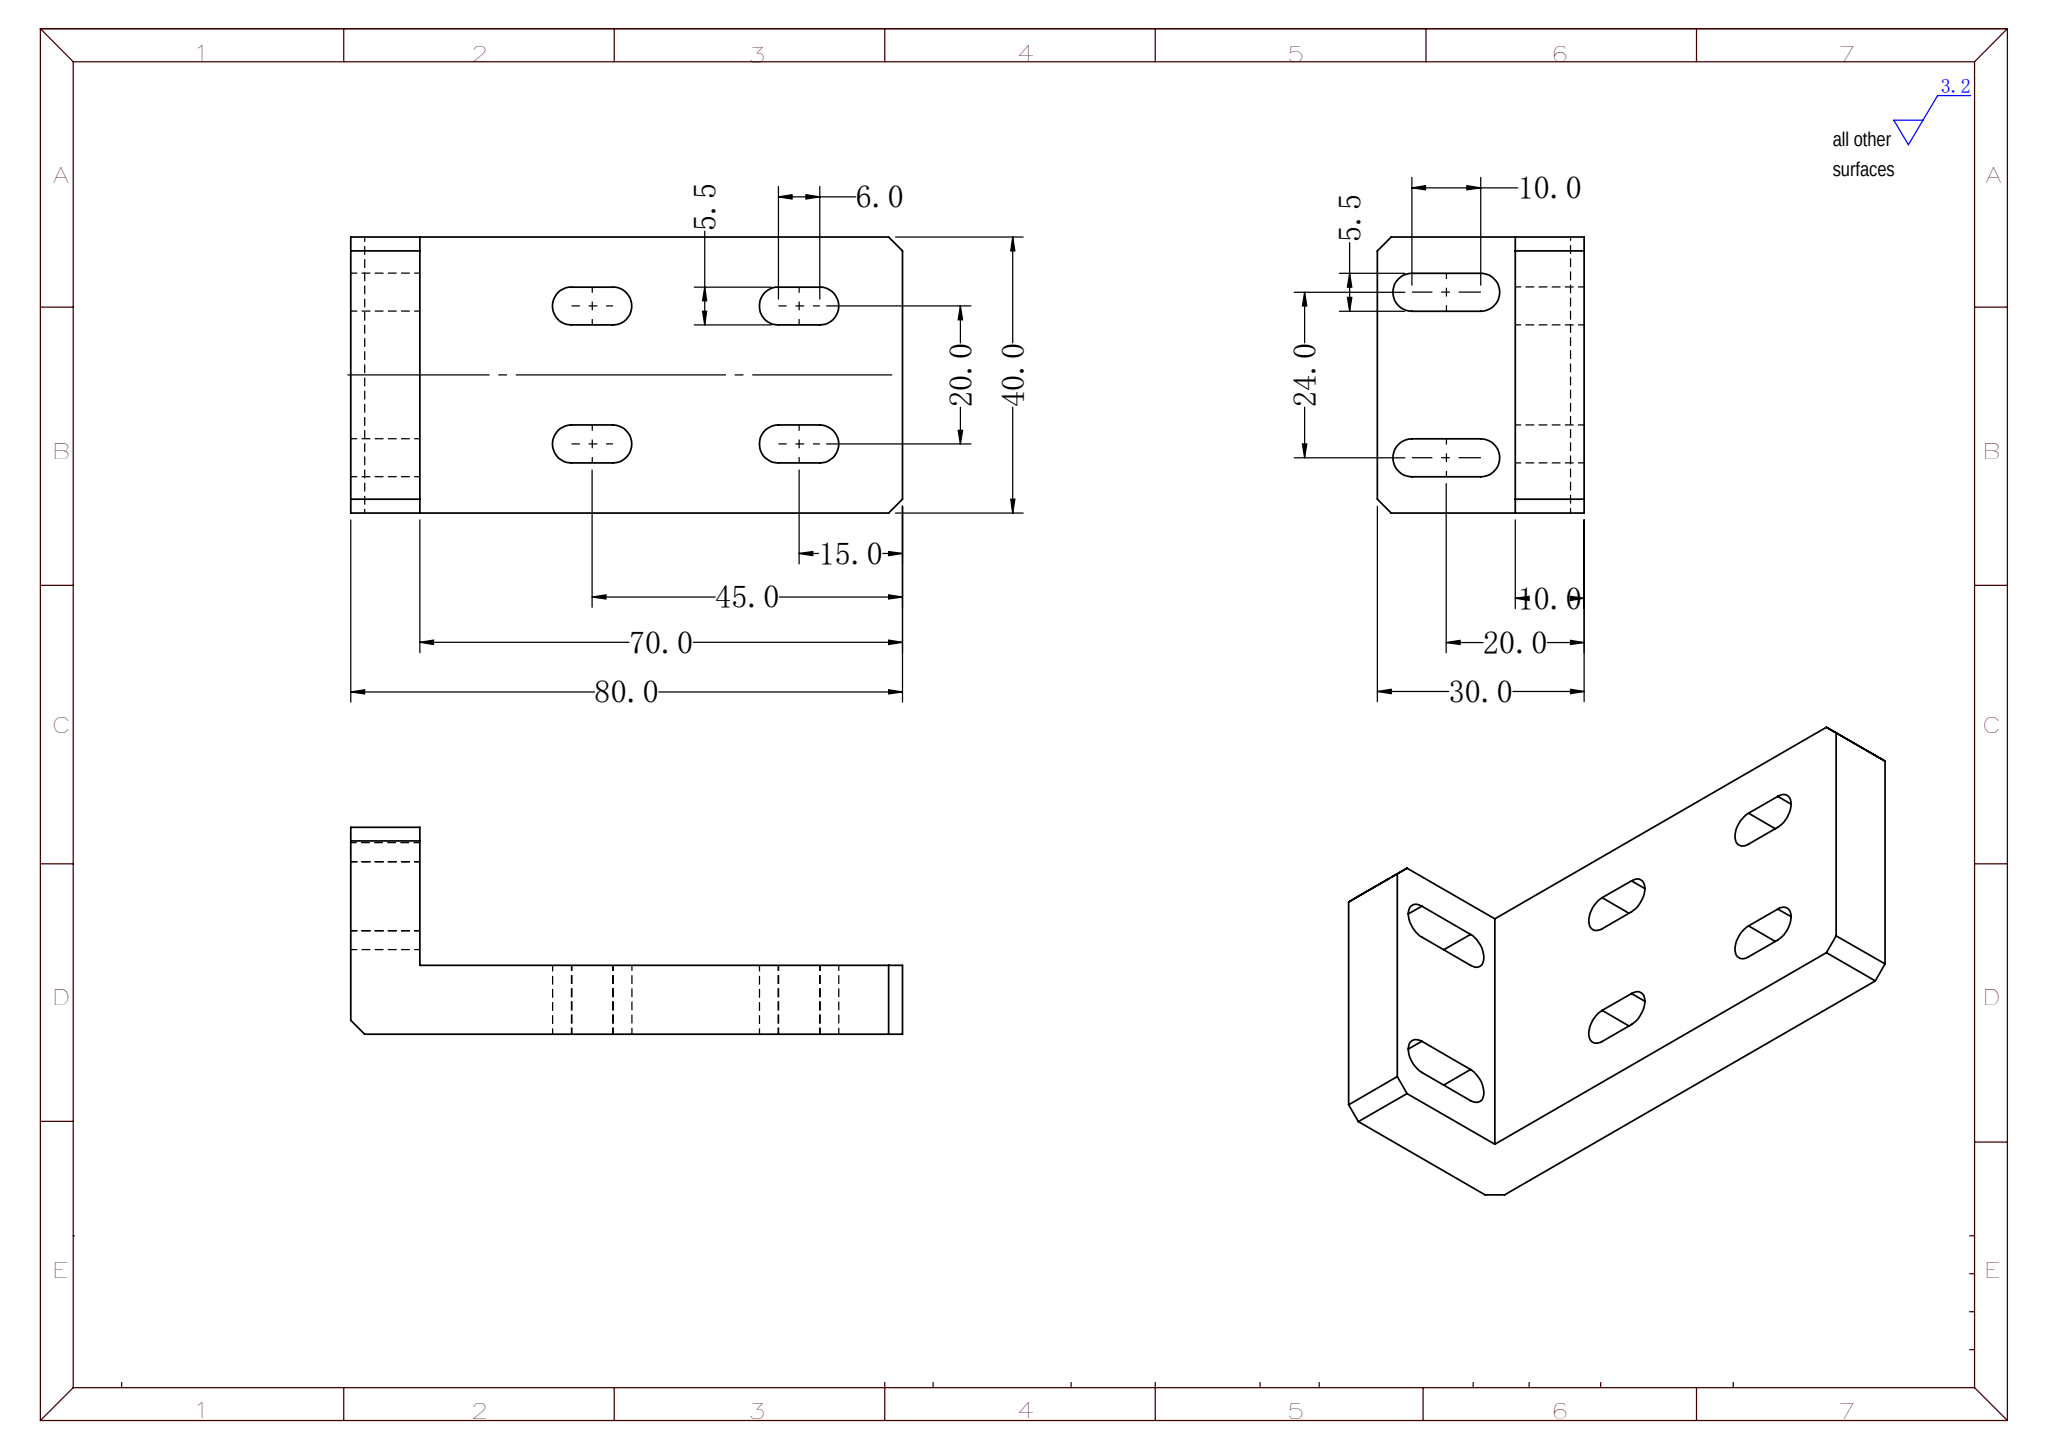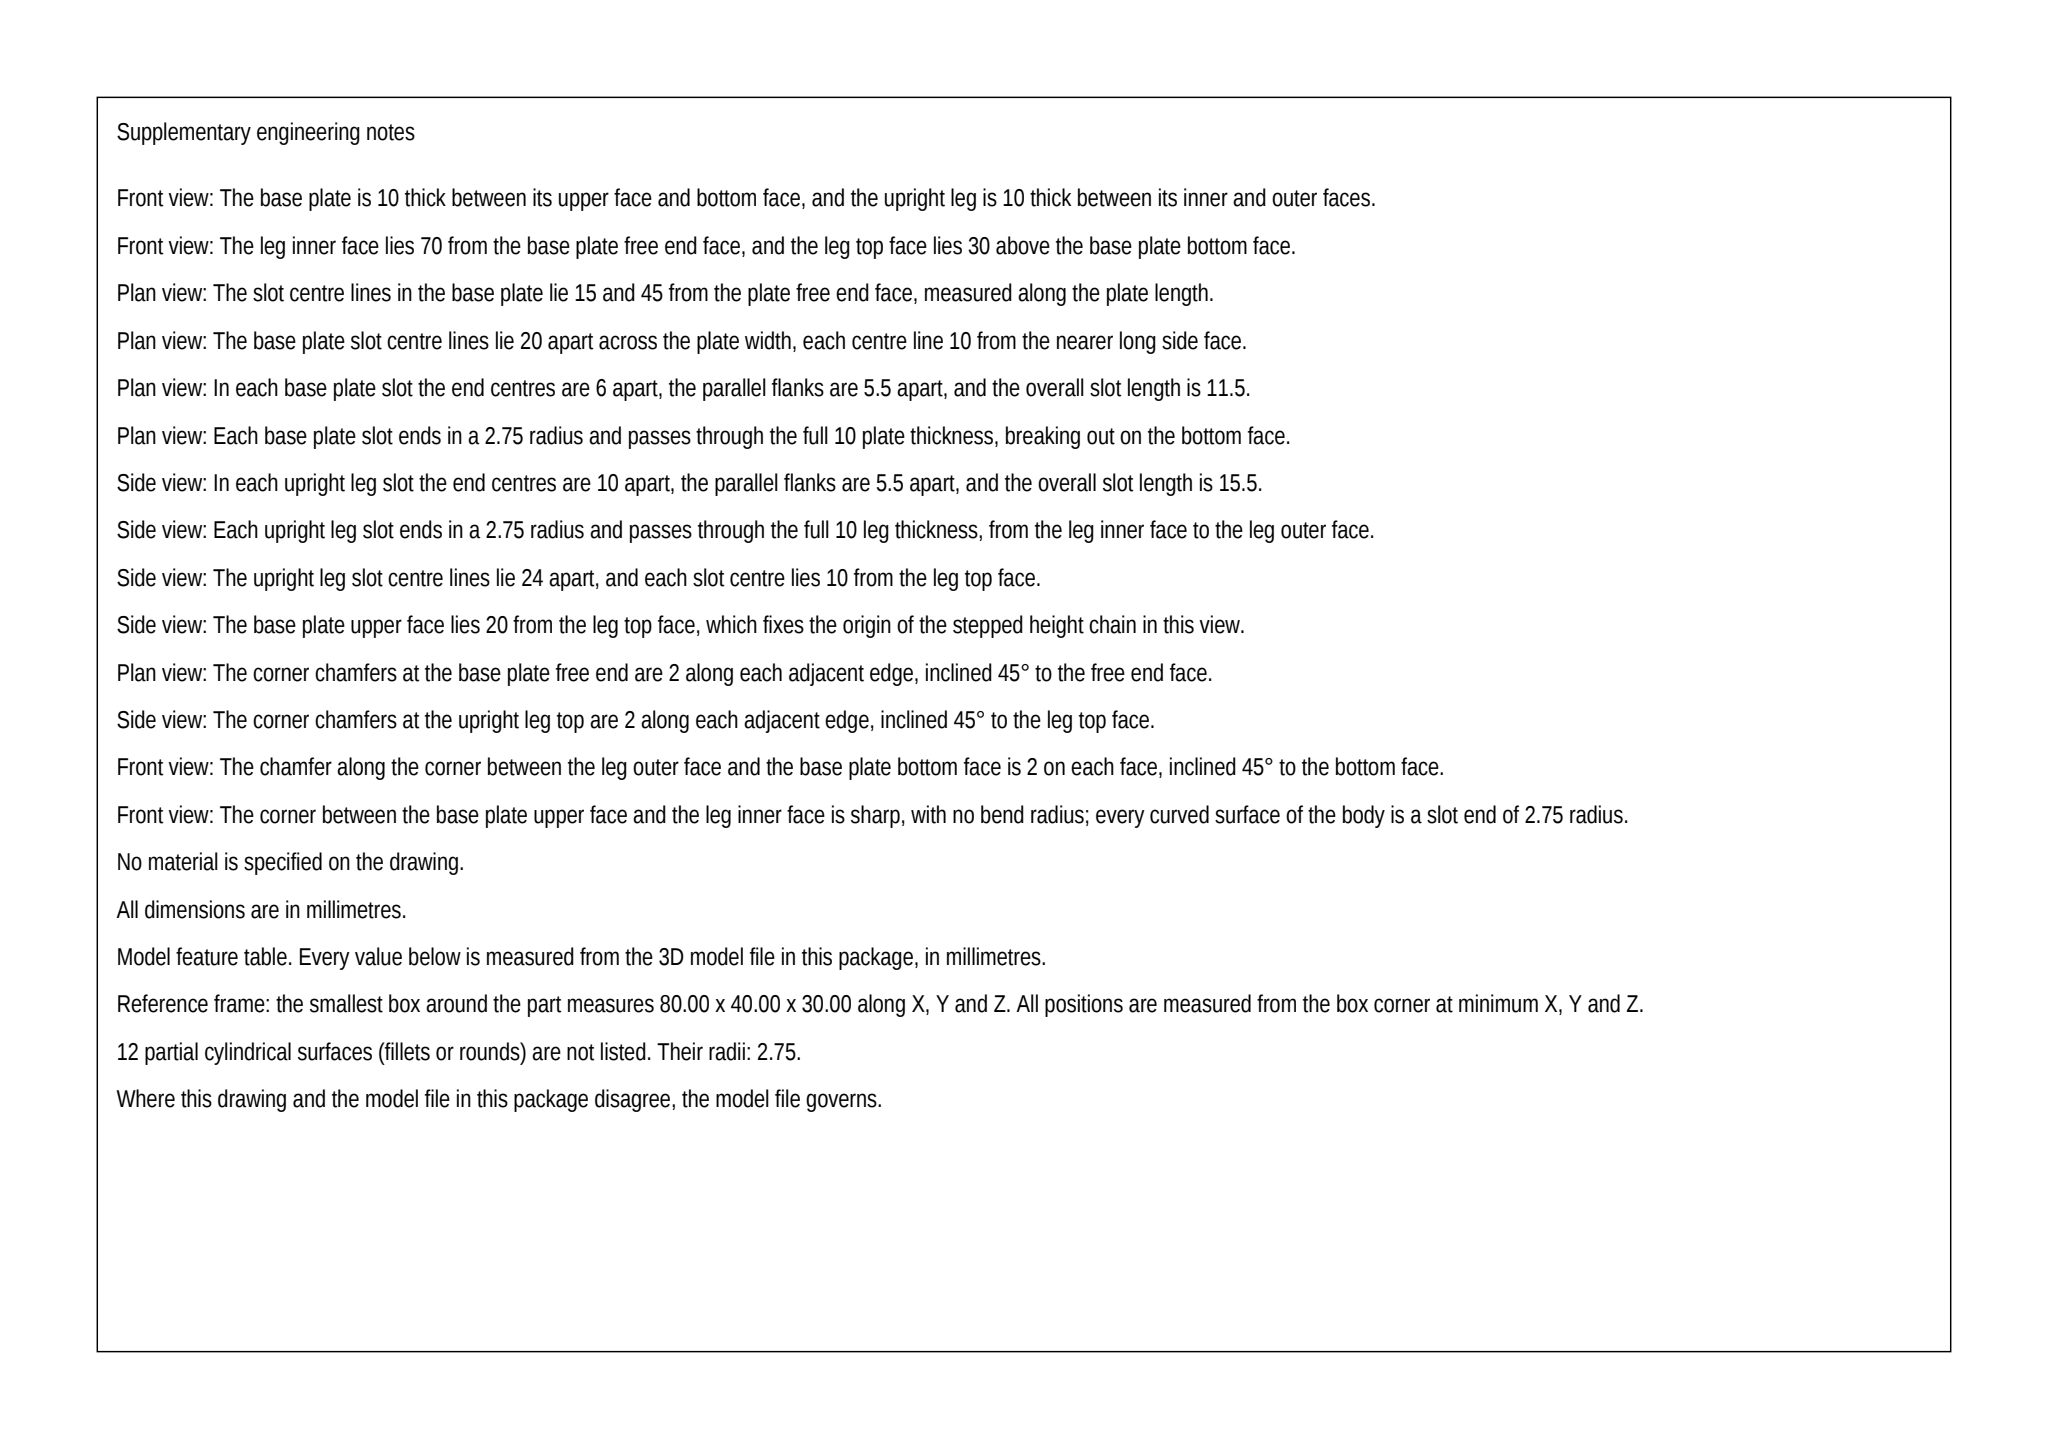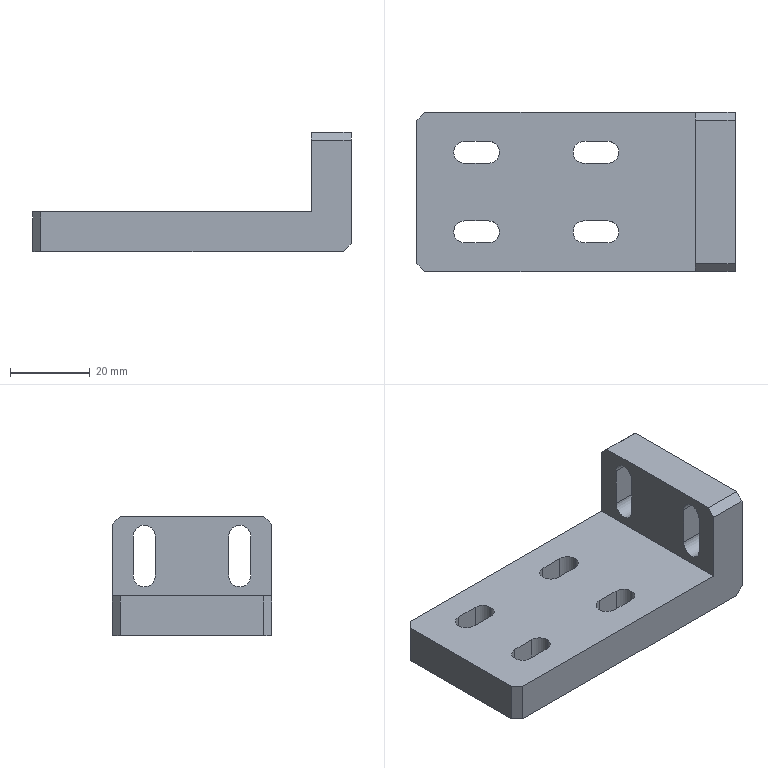Part | SolidWorks | mm | 1 solid | 43 faces | box 80 x 40 x 30 mm | volume 35995 mm3 | plane 25 | cylinder 18 | commonest cylinder face diameters 5.5 x18
Drawing notes:
ALL CORNERS C5 (5 x 45°) - PLATE END & UPRIGHT LEG | from the solid: BBox 80x40x30; corner cuts at x=0 plate end and leg top (z=30) are 45° planes, not in axis_planes list; measured leg 5 mm each side in TOP & SIDE views
build123d program:
from build123d import *

# Parameters (mm, degrees)
SKETCH1_W           = 80
SKETCH1_H           = 40
BOSS_EXTRUDE1_DEPTH = 15
SKETCH2_W           = 70
SKETCH2_H           = 20
CUT_EXTRUDE1_DEPTH  = 59.523
CUT_EXTRUDE2_DEPTH  = 75.33
CUT_EXTRUDE3_DEPTH  = 49.99
CHAMFER1_SIZE       = 2


with BuildPart() as part:
    # Sketch1 → Boss-Extrude1 (new, symmetric)
    with BuildSketch(Plane.XY):
        Rectangle(SKETCH1_W, SKETCH1_H)
    extrude(amount=BOSS_EXTRUDE1_DEPTH, both=True)

    # Sketch2 → Cut-Extrude1 (cut, through all)
    with BuildSketch(Plane(origin=(0, 20, 0), x_dir=(1, 0, 0), z_dir=(0, 1, 0))):
        with Locations((-5, -5)):
            Rectangle(SKETCH2_W, SKETCH2_H)
    extrude(amount=-CUT_EXTRUDE1_DEPTH, mode=Mode.SUBTRACT)

    # Sketch3 → Cut-Extrude2 (cut, through all)
    with BuildSketch(Plane.ZY.offset(-30)):
        with BuildLine():
            Line((0, 14.75), (10, 14.75))
            ThreePointArc((10, 14.75), (12.75, 12), (10, 9.25))
            Line((10, 9.25), (0, 9.25))
            ThreePointArc((0, 9.25), (-2.75, 12), (0, 14.75))
        make_face()
        with BuildLine():
            Line((0, -14.75), (10, -14.75))
            ThreePointArc((10, -14.75), (12.75, -12), (10, -9.25))
            Line((10, -9.25), (0, -9.25))
            ThreePointArc((0, -9.25), (-2.75, -12), (0, -14.75))
        make_face()
    extrude(amount=-CUT_EXTRUDE2_DEPTH, mode=Mode.SUBTRACT)

    # Sketch4 → Cut-Extrude3 (cut, through all)
    with BuildSketch(Plane.XY.offset(-5)):
        with BuildLine():
            Line((-28, 12.75), (-22, 12.75))
            ThreePointArc((-22, 12.75), (-19.25, 10), (-22, 7.25))
            Line((-22, 7.25), (-28, 7.25))
            ThreePointArc((-28, 7.25), (-30.75, 10), (-28, 12.75))
        make_face()
        with BuildLine():
            Line((2, 12.75), (8, 12.75))
            ThreePointArc((8, 12.75), (10.75, 10), (8, 7.25))
            Line((8, 7.25), (2, 7.25))
            ThreePointArc((2, 7.25), (-0.75, 10), (2, 12.75))
        make_face()
        with BuildLine():
            Line((-28, -12.75), (-22, -12.75))
            ThreePointArc((-22, -12.75), (-19.25, -10), (-22, -7.25))
            Line((-22, -7.25), (-28, -7.25))
            ThreePointArc((-28, -7.25), (-30.75, -10), (-28, -12.75))
        make_face()
        with BuildLine():
            Line((2, -12.75), (8, -12.75))
            ThreePointArc((8, -12.75), (10.75, -10), (8, -7.25))
            Line((8, -7.25), (2, -7.25))
            ThreePointArc((2, -7.25), (-0.75, -10), (2, -12.75))
        make_face()
    extrude(amount=-CUT_EXTRUDE3_DEPTH, mode=Mode.SUBTRACT)

    # Chamfer1
    chamfer1_edges = [part.edges().sort_by_distance(p)[0] for p in [
        (35, -20, 15),
        (-40, -20, -10),
        (-40, 20, -10),
        (40, 0, -15),
        (35, 20, 15),
    ]]
    chamfer(chamfer1_edges, length=CHAMFER1_SIZE)


solid = part.part